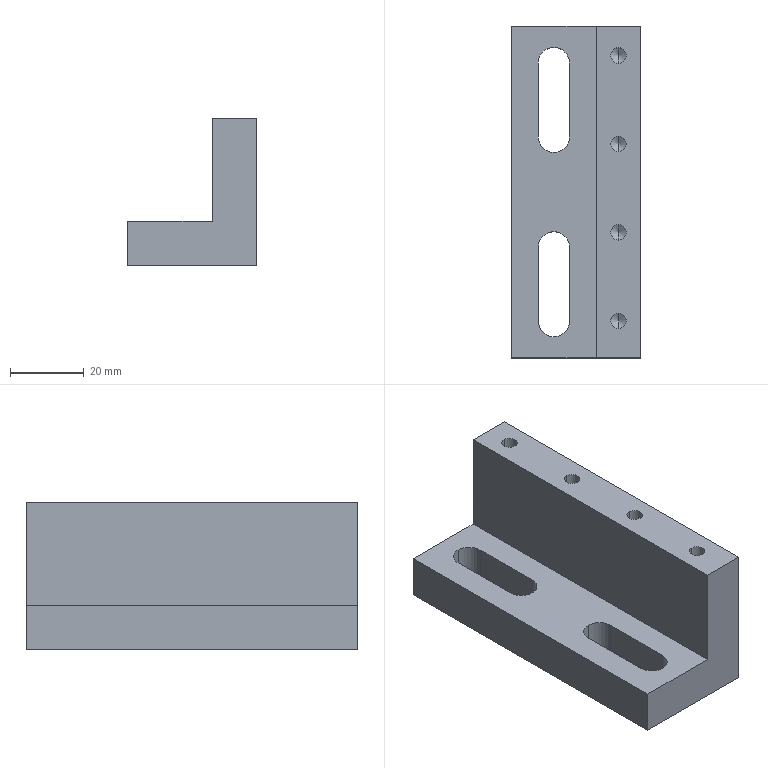Component | SolidWorks | DC-024-05-1 | 1 solid | 34 faces | box 35 x 90 x 40 mm | volume 61888 mm3 | cylinder 14 | plane 12 | cone 8 | commonest cylinder face diameters 4.2 x8 8.5 x6
build123d program:
from build123d import *

# Parameters (mm, degrees)
BOSS_EXTRUDE1_DEPTH   = 45
CUT_EXTRUDE1_DEPTH    = 80
M5_TAPPED_HOLE1_D     = 4.2
M5_TAPPED_HOLE1_DEPTH = 12.4
M5_TAPPED_HOLE1_TIP   = 1.262


with BuildPart() as part:
    # Sketch1 → Boss-Extrude1 (new, symmetric)
    with BuildSketch(Plane.XY):
        Polygon((0, 35), (0, 0), (40, 0), (40, 12), (12, 12), (12, 35), align=None)
    extrude(amount=BOSS_EXTRUDE1_DEPTH, both=True)

    # Sketch2 → Cut-Extrude1 (cut)
    with BuildSketch(Plane(origin=(12, 0, 0), x_dir=(0, 0, -1), z_dir=(1, 0, 0))):
        with BuildLine():
            Line((35, 19.25), (15, 19.25))
            ThreePointArc((15, 19.25), (10.75, 23.5), (15, 27.75))
            Line((15, 27.75), (35, 27.75))
            ThreePointArc((35, 27.75), (39.25, 23.5), (35, 19.25))
        make_face()
        with BuildLine():
            Line((-35, 19.25), (-15, 19.25))
            ThreePointArc((-15, 19.25), (-10.75, 23.5), (-15, 27.75))
            Line((-15, 27.75), (-35, 27.75))
            ThreePointArc((-35, 27.75), (-39.25, 23.5), (-35, 19.25))
        make_face()
    extrude(amount=-CUT_EXTRUDE1_DEPTH, mode=Mode.SUBTRACT)

    # M5 Tapped Hole1
    with Locations(Plane(origin=(40, 0, 0), x_dir=(0, 0, -1), z_dir=(1, 0, 0))):
        with Locations((37, 6), (13, 6), (-11, 6), (-35, 6)):
            Hole(M5_TAPPED_HOLE1_D / 2, depth=M5_TAPPED_HOLE1_DEPTH)
            with Locations((0, 0, -(M5_TAPPED_HOLE1_DEPTH + M5_TAPPED_HOLE1_TIP / 2))):  # 118° drill point
                Cone(0, M5_TAPPED_HOLE1_D / 2, M5_TAPPED_HOLE1_TIP, mode=Mode.SUBTRACT)


solid = part.part

# Placed as in the assembly
solid = solid.moved(Location((-78.633, -394.091, 13), (90, 0, 90)))
STEP:
#1=CARTESIAN_POINT('',(-3.332,-14.141,1.598));
#2=VERTEX_POINT('',#1);
#3=CARTESIAN_POINT('',(-3.332,-13.976,1.598));
#4=VERTEX_POINT('',#3);
#5=CARTESIAN_POINT('',(-3.332,-14.059,1.598));
#6=DIRECTION('',(-0.,-0.,1.));
#7=DIRECTION('',(0.,1.,0.));
#8=AXIS2_PLACEMENT_3D('',#5,#6,#7);
#9=CIRCLE('',#8,0.08268);
#10=EDGE_CURVE('',#2,#4,#9,.T.);
#11=ORIENTED_EDGE('',*,*,#10,.F.);
#12=CARTESIAN_POINT('',(-3.332,-14.141,2.087));
#13=VERTEX_POINT('',#12);
#14=CARTESIAN_POINT('',(-3.332,-14.141,2.087));
#15=DIRECTION('',(-0.,-0.,1.));
#16=VECTOR('',#15,39.37);
#17=LINE('',#14,#16);
#18=EDGE_CURVE('',#2,#13,#17,.T.);
#19=ORIENTED_EDGE('',*,*,#18,.T.);
#20=CARTESIAN_POINT('',(-3.332,-13.976,2.087));
#21=VERTEX_POINT('',#20);
#22=CARTESIAN_POINT('',(-3.332,-14.059,2.087));
#23=DIRECTION('',(-0.,-0.,1.));
#24=DIRECTION('',(0.,1.,0.));
#25=AXIS2_PLACEMENT_3D('',#22,#23,#24);
#26=CIRCLE('',#25,0.08268);
#27=EDGE_CURVE('',#13,#21,#26,.T.);
#28=ORIENTED_EDGE('',*,*,#27,.T.);
#29=CARTESIAN_POINT('',(-3.332,-13.976,2.087));
#30=DIRECTION('',(-0.,-0.,1.));
#31=VECTOR('',#30,39.37);
#32=LINE('',#29,#31);
#33=EDGE_CURVE('',#4,#21,#32,.T.);
#34=ORIENTED_EDGE('',*,*,#33,.F.);
#35=EDGE_LOOP('',(#11,#19,#28,#34));
#36=FACE_OUTER_BOUND('',#35,.T.);
#37=CARTESIAN_POINT('',(-3.332,-14.059,2.087));
#38=DIRECTION('',(-0.,-0.,1.));
#39=DIRECTION('',(0.,1.,0.));
#40=AXIS2_PLACEMENT_3D('',#37,#38,#39);
#41=CYLINDRICAL_SURFACE('',#40,0.08268);
#42=ADVANCED_FACE('',(#36),#41,.F.);
#43=CARTESIAN_POINT('',(-3.332,-14.059,1.549));
#44=VERTEX_POINT('',#43);
#45=CARTESIAN_POINT('',(-3.332,-13.976,1.598));
#46=DIRECTION('',(-0.,0.8572,0.515));
#47=VECTOR('',#46,39.37);
#48=LINE('',#45,#47);
#49=EDGE_CURVE('',#44,#4,#48,.T.);
#50=ORIENTED_EDGE('',*,*,#49,.F.);
#51=CARTESIAN_POINT('',(-3.332,-14.141,1.598));
#52=DIRECTION('',(0.,-0.8572,0.515));
#53=VECTOR('',#52,39.37);
#54=LINE('',#51,#53);
#55=EDGE_CURVE('',#44,#2,#54,.T.);
#56=ORIENTED_EDGE('',*,*,#55,.T.);
#57=ORIENTED_EDGE('',*,*,#10,.T.);
#58=EDGE_LOOP('',(#50,#56,#57));
#59=FACE_OUTER_BOUND('',#58,.T.);
#60=CARTESIAN_POINT('',(-3.332,-14.059,1.598));
#61=DIRECTION('',(-0.,-0.,1.));
#62=DIRECTION('',(0.,1.,0.));
#63=AXIS2_PLACEMENT_3D('',#60,#61,#62);
#64=CONICAL_SURFACE('',#63,0.08268,1.03);
#65=ADVANCED_FACE('',(#59),#64,.F.);
#66=CARTESIAN_POINT('',(-3.332,-15.086,1.598));
#67=VERTEX_POINT('',#66);
#68=CARTESIAN_POINT('',(-3.332,-14.921,1.598));
#69=VERTEX_POINT('',#68);
#70=CARTESIAN_POINT('',(-3.332,-15.004,1.598));
#71=DIRECTION('',(-0.,-0.,1.));
#72=DIRECTION('',(0.,1.,0.));
#73=AXIS2_PLACEMENT_3D('',#70,#71,#72);
#74=CIRCLE('',#73,0.08268);
#75=EDGE_CURVE('',#67,#69,#74,.T.);
#76=ORIENTED_EDGE('',*,*,#75,.F.);
#77=CARTESIAN_POINT('',(-3.332,-15.086,2.087));
#78=VERTEX_POINT('',#77);
#79=CARTESIAN_POINT('',(-3.332,-15.086,2.087));
#80=DIRECTION('',(-0.,-0.,1.));
#81=VECTOR('',#80,39.37);
#82=LINE('',#79,#81);
#83=EDGE_CURVE('',#67,#78,#82,.T.);
#84=ORIENTED_EDGE('',*,*,#83,.T.);
#85=CARTESIAN_POINT('',(-3.332,-14.921,2.087));
#86=VERTEX_POINT('',#85);
#87=CARTESIAN_POINT('',(-3.332,-15.004,2.087));
#88=DIRECTION('',(-0.,-0.,1.));
#89=DIRECTION('',(0.,1.,0.));
#90=AXIS2_PLACEMENT_3D('',#87,#88,#89);
#91=CIRCLE('',#90,0.08268);
#92=EDGE_CURVE('',#78,#86,#91,.T.);
#93=ORIENTED_EDGE('',*,*,#92,.T.);
#94=CARTESIAN_POINT('',(-3.332,-14.921,2.087));
#95=DIRECTION('',(-0.,-0.,1.));
#96=VECTOR('',#95,39.37);
#97=LINE('',#94,#96);
#98=EDGE_CURVE('',#69,#86,#97,.T.);
#99=ORIENTED_EDGE('',*,*,#98,.F.);
#100=EDGE_LOOP('',(#76,#84,#93,#99));
#101=FACE_OUTER_BOUND('',#100,.T.);
#102=CARTESIAN_POINT('',(-3.332,-15.004,2.087));
#103=DIRECTION('',(-0.,-0.,1.));
#104=DIRECTION('',(0.,1.,0.));
#105=AXIS2_PLACEMENT_3D('',#102,#103,#104);
#106=CYLINDRICAL_SURFACE('',#105,0.08268);
#107=ADVANCED_FACE('',(#101),#106,.F.);
#108=CARTESIAN_POINT('',(-3.332,-15.004,1.549));
#109=VERTEX_POINT('',#108);
#110=CARTESIAN_POINT('',(-3.332,-14.921,1.598));
#111=DIRECTION('',(-0.,0.8572,0.515));
#112=VECTOR('',#111,39.37);
#113=LINE('',#110,#112);
#114=EDGE_CURVE('',#109,#69,#113,.T.);
#115=ORIENTED_EDGE('',*,*,#114,.F.);
#116=CARTESIAN_POINT('',(-3.332,-15.086,1.598));
#117=DIRECTION('',(0.,-0.8572,0.515));
#118=VECTOR('',#117,39.37);
#119=LINE('',#116,#118);
#120=EDGE_CURVE('',#109,#67,#119,.T.);
#121=ORIENTED_EDGE('',*,*,#120,.T.);
#122=ORIENTED_EDGE('',*,*,#75,.T.);
#123=EDGE_LOOP('',(#115,#121,#122));
#124=FACE_OUTER_BOUND('',#123,.T.);
#125=CARTESIAN_POINT('',(-3.332,-15.004,1.598));
#126=DIRECTION('',(-0.,-0.,1.));
#127=DIRECTION('',(0.,1.,0.));
#128=AXIS2_PLACEMENT_3D('',#125,#126,#127);
#129=CONICAL_SURFACE('',#128,0.08268,1.03);
#130=ADVANCED_FACE('',(#124),#129,.F.);
#131=CARTESIAN_POINT('',(-3.332,-16.031,1.598));
#132=VERTEX_POINT('',#131);
#133=CARTESIAN_POINT('',(-3.332,-15.866,1.598));
#134=VERTEX_POINT('',#133);
#135=CARTESIAN_POINT('',(-3.332,-15.948,1.598));
#136=DIRECTION('',(-0.,-0.,1.));
#137=DIRECTION('',(0.,1.,0.));
#138=AXIS2_PLACEMENT_3D('',#135,#136,#137);
#139=CIRCLE('',#138,0.08268);
#140=EDGE_CURVE('',#132,#134,#139,.T.);
#141=ORIENTED_EDGE('',*,*,#140,.F.);
#142=CARTESIAN_POINT('',(-3.332,-16.031,2.087));
#143=VERTEX_POINT('',#142);
#144=CARTESIAN_POINT('',(-3.332,-16.031,2.087));
#145=DIRECTION('',(-0.,-0.,1.));
#146=VECTOR('',#145,39.37);
#147=LINE('',#144,#146);
#148=EDGE_CURVE('',#132,#143,#147,.T.);
#149=ORIENTED_EDGE('',*,*,#148,.T.);
#150=CARTESIAN_POINT('',(-3.332,-15.866,2.087));
#151=VERTEX_POINT('',#150);
#152=CARTESIAN_POINT('',(-3.332,-15.948,2.087));
#153=DIRECTION('',(-0.,-0.,1.));
#154=DIRECTION('',(0.,1.,0.));
#155=AXIS2_PLACEMENT_3D('',#152,#153,#154);
#156=CIRCLE('',#155,0.08268);
#157=EDGE_CURVE('',#143,#151,#156,.T.);
#158=ORIENTED_EDGE('',*,*,#157,.T.);
#159=CARTESIAN_POINT('',(-3.332,-15.866,2.087));
#160=DIRECTION('',(-0.,-0.,1.));
#161=VECTOR('',#160,39.37);
#162=LINE('',#159,#161);
#163=EDGE_CURVE('',#134,#151,#162,.T.);
#164=ORIENTED_EDGE('',*,*,#163,.F.);
#165=EDGE_LOOP('',(#141,#149,#158,#164));
#166=FACE_OUTER_BOUND('',#165,.T.);
#167=CARTESIAN_POINT('',(-3.332,-15.948,2.087));
#168=DIRECTION('',(-0.,-0.,1.));
#169=DIRECTION('',(0.,1.,0.));
#170=AXIS2_PLACEMENT_3D('',#167,#168,#169);
#171=CYLINDRICAL_SURFACE('',#170,0.08268);
#172=ADVANCED_FACE('',(#166),#171,.F.);
#173=CARTESIAN_POINT('',(-3.332,-15.948,1.549));
#174=VERTEX_POINT('',#173);
#175=CARTESIAN_POINT('',(-3.332,-15.866,1.598));
#176=DIRECTION('',(-0.,0.8572,0.515));
#177=VECTOR('',#176,39.37);
#178=LINE('',#175,#177);
#179=EDGE_CURVE('',#174,#134,#178,.T.);
#180=ORIENTED_EDGE('',*,*,#179,.F.);
#181=CARTESIAN_POINT('',(-3.332,-16.031,1.598));
#182=DIRECTION('',(0.,-0.8572,0.515));
#183=VECTOR('',#182,39.37);
#184=LINE('',#181,#183);
#185=EDGE_CURVE('',#174,#132,#184,.T.);
#186=ORIENTED_EDGE('',*,*,#185,.T.);
#187=ORIENTED_EDGE('',*,*,#140,.T.);
#188=EDGE_LOOP('',(#180,#186,#187));
#189=FACE_OUTER_BOUND('',#188,.T.);
#190=CARTESIAN_POINT('',(-3.332,-15.948,1.598));
#191=DIRECTION('',(-0.,-0.,1.));
#192=DIRECTION('',(0.,1.,0.));
#193=AXIS2_PLACEMENT_3D('',#190,#191,#192);
#194=CONICAL_SURFACE('',#193,0.08268,1.03);
#195=ADVANCED_FACE('',(#189),#194,.F.);
#196=CARTESIAN_POINT('',(-3.332,-16.976,1.598));
#197=VERTEX_POINT('',#196);
#198=CARTESIAN_POINT('',(-3.332,-16.811,1.598));
#199=VERTEX_POINT('',#198);
#200=CARTESIAN_POINT('',(-3.332,-16.893,1.598));
#201=DIRECTION('',(-0.,-0.,1.));
#202=DIRECTION('',(0.,1.,0.));
#203=AXIS2_PLACEMENT_3D('',#200,#201,#202);
#204=CIRCLE('',#203,0.08268);
#205=EDGE_CURVE('',#197,#199,#204,.T.);
#206=ORIENTED_EDGE('',*,*,#205,.F.);
#207=CARTESIAN_POINT('',(-3.332,-16.976,2.087));
#208=VERTEX_POINT('',#207);
#209=CARTESIAN_POINT('',(-3.332,-16.976,2.087));
#210=DIRECTION('',(-0.,-0.,1.));
#211=VECTOR('',#210,39.37);
#212=LINE('',#209,#211);
#213=EDGE_CURVE('',#197,#208,#212,.T.);
#214=ORIENTED_EDGE('',*,*,#213,.T.);
#215=CARTESIAN_POINT('',(-3.332,-16.811,2.087));
#216=VERTEX_POINT('',#215);
#217=CARTESIAN_POINT('',(-3.332,-16.893,2.087));
#218=DIRECTION('',(-0.,-0.,1.));
#219=DIRECTION('',(0.,1.,0.));
#220=AXIS2_PLACEMENT_3D('',#217,#218,#219);
#221=CIRCLE('',#220,0.08268);
#222=EDGE_CURVE('',#208,#216,#221,.T.);
#223=ORIENTED_EDGE('',*,*,#222,.T.);
#224=CARTESIAN_POINT('',(-3.332,-16.811,2.087));
#225=DIRECTION('',(-0.,-0.,1.));
#226=VECTOR('',#225,39.37);
#227=LINE('',#224,#226);
#228=EDGE_CURVE('',#199,#216,#227,.T.);
#229=ORIENTED_EDGE('',*,*,#228,.F.);
#230=EDGE_LOOP('',(#206,#214,#223,#229));
#231=FACE_OUTER_BOUND('',#230,.T.);
#232=CARTESIAN_POINT('',(-3.332,-16.893,2.087));
#233=DIRECTION('',(-0.,-0.,1.));
#234=DIRECTION('',(0.,1.,0.));
#235=AXIS2_PLACEMENT_3D('',#232,#233,#234);
#236=CYLINDRICAL_SURFACE('',#235,0.08268);
#237=ADVANCED_FACE('',(#231),#236,.F.);
#238=CARTESIAN_POINT('',(-3.332,-16.893,1.549));
#239=VERTEX_POINT('',#238);
#240=CARTESIAN_POINT('',(-3.332,-16.811,1.598));
#241=DIRECTION('',(-0.,0.8572,0.515));
#242=VECTOR('',#241,39.37);
#243=LINE('',#240,#242);
#244=EDGE_CURVE('',#239,#199,#243,.T.);
#245=ORIENTED_EDGE('',*,*,#244,.F.);
#246=CARTESIAN_POINT('',(-3.332,-16.976,1.598));
#247=DIRECTION('',(0.,-0.8572,0.515));
#248=VECTOR('',#247,39.37);
#249=LINE('',#246,#248);
#250=EDGE_CURVE('',#239,#197,#249,.T.);
#251=ORIENTED_EDGE('',*,*,#250,.T.);
#252=ORIENTED_EDGE('',*,*,#205,.T.);
#253=EDGE_LOOP('',(#245,#251,#252));
#254=FACE_OUTER_BOUND('',#253,.T.);
#255=CARTESIAN_POINT('',(-3.332,-16.893,1.598));
#256=DIRECTION('',(-0.,-0.,1.));
#257=DIRECTION('',(0.,1.,0.));
#258=AXIS2_PLACEMENT_3D('',#255,#256,#257);
#259=CONICAL_SURFACE('',#258,0.08268,1.03);
#260=ADVANCED_FACE('',(#254),#259,.F.);
#261=CARTESIAN_POINT('',(-4.021,-13.97,0.5118));
#262=VERTEX_POINT('',#261);
#263=CARTESIAN_POINT('',(-4.188,-14.137,0.5118));
#264=VERTEX_POINT('',#263);
#265=CARTESIAN_POINT('',(-4.021,-14.137,0.5118));
#266=DIRECTION('',(-0.,-0.,1.));
#267=DIRECTION('',(-1.,0.,0.));
#268=AXIS2_PLACEMENT_3D('',#265,#266,#267);
#269=CIRCLE('',#268,0.1673);
#270=EDGE_CURVE('',#262,#264,#269,.T.);
#271=ORIENTED_EDGE('',*,*,#270,.F.);
#272=CARTESIAN_POINT('',(-4.021,-13.97,0.9843));
#273=VERTEX_POINT('',#272);
#274=CARTESIAN_POINT('',(-4.021,-13.97,-2.165));
#275=DIRECTION('',(-0.,-0.,1.));
#276=VECTOR('',#275,39.37);
#277=LINE('',#274,#276);
#278=EDGE_CURVE('',#262,#273,#277,.T.);
#279=ORIENTED_EDGE('',*,*,#278,.T.);
#280=CARTESIAN_POINT('',(-4.188,-14.137,0.9843));
#281=VERTEX_POINT('',#280);
#282=CARTESIAN_POINT('',(-4.021,-14.137,0.9843));
#283=DIRECTION('',(-0.,-0.,1.));
#284=DIRECTION('',(0.,1.,0.));
#285=AXIS2_PLACEMENT_3D('',#282,#283,#284);
#286=CIRCLE('',#285,0.1673);
#287=EDGE_CURVE('',#273,#281,#286,.T.);
#288=ORIENTED_EDGE('',*,*,#287,.T.);
#289=CARTESIAN_POINT('',(-4.188,-14.137,-2.165));
#290=DIRECTION('',(-0.,-0.,1.));
#291=VECTOR('',#290,39.37);
#292=LINE('',#289,#291);
#293=EDGE_CURVE('',#264,#281,#292,.T.);
#294=ORIENTED_EDGE('',*,*,#293,.F.);
#295=EDGE_LOOP('',(#271,#279,#288,#294));
#296=FACE_OUTER_BOUND('',#295,.T.);
#297=CARTESIAN_POINT('',(-4.021,-14.137,-2.165));
#298=DIRECTION('',(-0.,-0.,1.));
#299=DIRECTION('',(0.,1.,0.));
#300=AXIS2_PLACEMENT_3D('',#297,#298,#299);
#301=CYLINDRICAL_SURFACE('',#300,0.1673);
#302=ADVANCED_FACE('',(#296),#301,.F.);
#303=CARTESIAN_POINT('',(-4.021,-15.939,0.5118));
#304=VERTEX_POINT('',#303);
#305=CARTESIAN_POINT('',(-4.188,-16.106,0.5118));
#306=VERTEX_POINT('',#305);
#307=CARTESIAN_POINT('',(-4.021,-16.106,0.5118));
#308=DIRECTION('',(-0.,-0.,1.));
#309=DIRECTION('',(-1.,0.,0.));
#310=AXIS2_PLACEMENT_3D('',#307,#308,#309);
#311=CIRCLE('',#310,0.1673);
#312=EDGE_CURVE('',#304,#306,#311,.T.);
#313=ORIENTED_EDGE('',*,*,#312,.F.);
#314=CARTESIAN_POINT('',(-4.021,-15.939,0.9843));
#315=VERTEX_POINT('',#314);
#316=CARTESIAN_POINT('',(-4.021,-15.939,-2.165));
#317=DIRECTION('',(-0.,-0.,1.));
#318=VECTOR('',#317,39.37);
#319=LINE('',#316,#318);
#320=EDGE_CURVE('',#304,#315,#319,.T.);
#321=ORIENTED_EDGE('',*,*,#320,.T.);
#322=CARTESIAN_POINT('',(-4.188,-16.106,0.9843));
#323=VERTEX_POINT('',#322);
#324=CARTESIAN_POINT('',(-4.021,-16.106,0.9843));
#325=DIRECTION('',(-0.,-0.,1.));
#326=DIRECTION('',(0.,-1.,0.));
#327=AXIS2_PLACEMENT_3D('',#324,#325,#326);
#328=CIRCLE('',#327,0.1673);
#329=EDGE_CURVE('',#315,#323,#328,.T.);
#330=ORIENTED_EDGE('',*,*,#329,.T.);
#331=CARTESIAN_POINT('',(-4.188,-16.106,-2.165));
#332=DIRECTION('',(-0.,-0.,1.));
#333=VECTOR('',#332,39.37);
#334=LINE('',#331,#333);
#335=EDGE_CURVE('',#306,#323,#334,.T.);
#336=ORIENTED_EDGE('',*,*,#335,.F.);
#337=EDGE_LOOP('',(#313,#321,#330,#336));
#338=FACE_OUTER_BOUND('',#337,.T.);
#339=CARTESIAN_POINT('',(-4.021,-16.106,-2.165));
#340=DIRECTION('',(-0.,-0.,1.));
#341=DIRECTION('',(0.,1.,0.));
#342=AXIS2_PLACEMENT_3D('',#339,#340,#341);
#343=CYLINDRICAL_SURFACE('',#342,0.1673);
#344=ADVANCED_FACE('',(#338),#343,.F.);
#345=CARTESIAN_POINT('',(-4.474,-13.744,0.9843));
#346=VERTEX_POINT('',#345);
#347=CARTESIAN_POINT('',(-4.474,-13.744,0.5118));
#348=VERTEX_POINT('',#347);
#349=CARTESIAN_POINT('',(-4.474,-13.744,0.5118));
#350=DIRECTION('',(0.,0.,-1.));
#351=VECTOR('',#350,39.37);
#352=LINE('',#349,#351);
#353=EDGE_CURVE('',#346,#348,#352,.T.);
#354=ORIENTED_EDGE('',*,*,#353,.T.);
#355=CARTESIAN_POINT('',(-4.474,-17.287,0.5118));
#356=VERTEX_POINT('',#355);
#357=CARTESIAN_POINT('',(-4.474,-17.287,0.5118));
#358=DIRECTION('',(-0.,1.,0.));
#359=VECTOR('',#358,39.37);
#360=LINE('',#357,#359);
#361=EDGE_CURVE('',#356,#348,#360,.T.);
#362=ORIENTED_EDGE('',*,*,#361,.F.);
#363=CARTESIAN_POINT('',(-4.474,-17.287,0.9843));
#364=VERTEX_POINT('',#363);
#365=CARTESIAN_POINT('',(-4.474,-17.287,0.5118));
#366=DIRECTION('',(0.,0.,-1.));
#367=VECTOR('',#366,39.37);
#368=LINE('',#365,#367);
#369=EDGE_CURVE('',#364,#356,#368,.T.);
#370=ORIENTED_EDGE('',*,*,#369,.F.);
#371=CARTESIAN_POINT('',(-4.474,-17.287,0.9843));
#372=DIRECTION('',(-0.,1.,0.));
#373=VECTOR('',#372,39.37);
#374=LINE('',#371,#373);
#375=EDGE_CURVE('',#364,#346,#374,.T.);
#376=ORIENTED_EDGE('',*,*,#375,.T.);
#377=EDGE_LOOP('',(#354,#362,#370,#376));
#378=FACE_OUTER_BOUND('',#377,.T.);
#379=CARTESIAN_POINT('',(-4.474,-17.287,0.5118));
#380=DIRECTION('',(1.,0.,0.));
#381=DIRECTION('',(-0.,1.,0.));
#382=AXIS2_PLACEMENT_3D('',#379,#380,#381);
#383=PLANE('',#382);
#384=ADVANCED_FACE('',(#378),#383,.F.);
#385=CARTESIAN_POINT('',(-3.854,-14.925,0.5118));
#386=VERTEX_POINT('',#385);
#387=CARTESIAN_POINT('',(-3.854,-14.137,0.5118));
#388=VERTEX_POINT('',#387);
#389=CARTESIAN_POINT('',(-3.854,-17.287,0.5118));
#390=DIRECTION('',(-0.,1.,0.));
#391=VECTOR('',#390,39.37);
#392=LINE('',#389,#391);
#393=EDGE_CURVE('',#386,#388,#392,.T.);
#394=ORIENTED_EDGE('',*,*,#393,.T.);
#395=CARTESIAN_POINT('',(-4.021,-14.137,0.5118));
#396=DIRECTION('',(-0.,-0.,1.));
#397=DIRECTION('',(-1.,0.,0.));
#398=AXIS2_PLACEMENT_3D('',#395,#396,#397);
#399=CIRCLE('',#398,0.1673);
#400=EDGE_CURVE('',#388,#262,#399,.T.);
#401=ORIENTED_EDGE('',*,*,#400,.T.);
#402=ORIENTED_EDGE('',*,*,#270,.T.);
#403=CARTESIAN_POINT('',(-4.188,-14.925,0.5118));
#404=VERTEX_POINT('',#403);
#405=CARTESIAN_POINT('',(-4.188,-17.287,0.5118));
#406=DIRECTION('',(0.,-1.,0.));
#407=VECTOR('',#406,39.37);
#408=LINE('',#405,#407);
#409=EDGE_CURVE('',#264,#404,#408,.T.);
#410=ORIENTED_EDGE('',*,*,#409,.T.);
#411=CARTESIAN_POINT('',(-4.021,-14.925,0.5118));
#412=DIRECTION('',(-0.,-0.,1.));
#413=DIRECTION('',(-1.,0.,0.));
#414=AXIS2_PLACEMENT_3D('',#411,#412,#413);
#415=CIRCLE('',#414,0.1673);
#416=EDGE_CURVE('',#404,#386,#415,.T.);
#417=ORIENTED_EDGE('',*,*,#416,.T.);
#418=EDGE_LOOP('',(#394,#401,#402,#410,#417));
#419=FACE_BOUND('',#418,.T.);
#420=CARTESIAN_POINT('',(-4.188,-16.893,0.5118));
#421=VERTEX_POINT('',#420);
#422=CARTESIAN_POINT('',(-4.188,-17.287,0.5118));
#423=DIRECTION('',(0.,-1.,0.));
#424=VECTOR('',#423,39.37);
#425=LINE('',#422,#424);
#426=EDGE_CURVE('',#306,#421,#425,.T.);
#427=ORIENTED_EDGE('',*,*,#426,.T.);
#428=CARTESIAN_POINT('',(-3.854,-16.893,0.5118));
#429=VERTEX_POINT('',#428);
#430=CARTESIAN_POINT('',(-4.021,-16.893,0.5118));
#431=DIRECTION('',(-0.,-0.,1.));
#432=DIRECTION('',(-1.,0.,0.));
#433=AXIS2_PLACEMENT_3D('',#430,#431,#432);
#434=CIRCLE('',#433,0.1673);
#435=EDGE_CURVE('',#421,#429,#434,.T.);
#436=ORIENTED_EDGE('',*,*,#435,.T.);
#437=CARTESIAN_POINT('',(-3.854,-16.106,0.5118));
#438=VERTEX_POINT('',#437);
#439=CARTESIAN_POINT('',(-3.854,-17.287,0.5118));
#440=DIRECTION('',(-0.,1.,0.));
#441=VECTOR('',#440,39.37);
#442=LINE('',#439,#441);
#443=EDGE_CURVE('',#429,#438,#442,.T.);
#444=ORIENTED_EDGE('',*,*,#443,.T.);
#445=CARTESIAN_POINT('',(-4.021,-16.106,0.5118));
#446=DIRECTION('',(-0.,-0.,1.));
#447=DIRECTION('',(-1.,0.,0.));
#448=AXIS2_PLACEMENT_3D('',#445,#446,#447);
#449=CIRCLE('',#448,0.1673);
#450=EDGE_CURVE('',#438,#304,#449,.T.);
#451=ORIENTED_EDGE('',*,*,#450,.T.);
#452=ORIENTED_EDGE('',*,*,#312,.T.);
#453=EDGE_LOOP('',(#427,#436,#444,#451,#452));
#454=FACE_BOUND('',#453,.T.);
#455=CARTESIAN_POINT('',(-3.096,-13.744,0.5118));
#456=VERTEX_POINT('',#455);
#457=CARTESIAN_POINT('',(-4.474,-13.744,0.5118));
#458=DIRECTION('',(1.,0.,0.));
#459=VECTOR('',#458,39.37);
#460=LINE('',#457,#459);
#461=EDGE_CURVE('',#348,#456,#460,.T.);
#462=ORIENTED_EDGE('',*,*,#461,.T.);
#463=CARTESIAN_POINT('',(-3.096,-17.287,0.5118));
#464=VERTEX_POINT('',#463);
#465=CARTESIAN_POINT('',(-3.096,-17.287,0.5118));
#466=DIRECTION('',(-0.,1.,0.));
#467=VECTOR('',#466,39.37);
#468=LINE('',#465,#467);
#469=EDGE_CURVE('',#464,#456,#468,.T.);
#470=ORIENTED_EDGE('',*,*,#469,.F.);
#471=CARTESIAN_POINT('',(-4.474,-17.287,0.5118));
#472=DIRECTION('',(1.,0.,0.));
#473=VECTOR('',#472,39.37);
#474=LINE('',#471,#473);
#475=EDGE_CURVE('',#356,#464,#474,.T.);
#476=ORIENTED_EDGE('',*,*,#475,.F.);
#477=ORIENTED_EDGE('',*,*,#361,.T.);
#478=EDGE_LOOP('',(#462,#470,#476,#477));
#479=FACE_OUTER_BOUND('',#478,.T.);
#480=CARTESIAN_POINT('',(-4.474,-17.287,0.5118));
#481=DIRECTION('',(-0.,-0.,1.));
#482=DIRECTION('',(-1.,-0.,-0.));
#483=AXIS2_PLACEMENT_3D('',#480,#481,#482);
#484=PLANE('',#483);
#485=ADVANCED_FACE('',(#419,#454,#479),#484,.F.);
#486=CARTESIAN_POINT('',(-3.096,-13.744,2.087));
#487=VERTEX_POINT('',#486);
#488=CARTESIAN_POINT('',(-3.096,-13.744,0.5118));
#489=DIRECTION('',(-0.,-0.,1.));
#490=VECTOR('',#489,39.37);
#491=LINE('',#488,#490);
#492=EDGE_CURVE('',#456,#487,#491,.T.);
#493=ORIENTED_EDGE('',*,*,#492,.T.);
#494=CARTESIAN_POINT('',(-3.096,-17.287,2.087));
#495=VERTEX_POINT('',#494);
#496=CARTESIAN_POINT('',(-3.096,-17.287,2.087));
#497=DIRECTION('',(-0.,1.,0.));
#498=VECTOR('',#497,39.37);
#499=LINE('',#496,#498);
#500=EDGE_CURVE('',#495,#487,#499,.T.);
#501=ORIENTED_EDGE('',*,*,#500,.F.);
#502=CARTESIAN_POINT('',(-3.096,-17.287,0.5118));
#503=DIRECTION('',(-0.,-0.,1.));
#504=VECTOR('',#503,39.37);
#505=LINE('',#502,#504);
#506=EDGE_CURVE('',#464,#495,#505,.T.);
#507=ORIENTED_EDGE('',*,*,#506,.F.);
#508=ORIENTED_EDGE('',*,*,#469,.T.);
#509=EDGE_LOOP('',(#493,#501,#507,#508));
#510=FACE_OUTER_BOUND('',#509,.T.);
#511=CARTESIAN_POINT('',(-3.096,-17.287,0.5118));
#512=DIRECTION('',(-1.,-0.,-0.));
#513=DIRECTION('',(0.,-1.,0.));
#514=AXIS2_PLACEMENT_3D('',#511,#512,#513);
#515=PLANE('',#514);
#516=ADVANCED_FACE('',(#510),#515,.F.);
#517=CARTESIAN_POINT('',(-3.332,-14.059,2.087));
#518=DIRECTION('',(-0.,-0.,1.));
#519=DIRECTION('',(0.,1.,0.));
#520=AXIS2_PLACEMENT_3D('',#517,#518,#519);
#521=CIRCLE('',#520,0.08268);
#522=EDGE_CURVE('',#21,#13,#521,.T.);
#523=ORIENTED_EDGE('',*,*,#522,.F.);
#524=ORIENTED_EDGE('',*,*,#27,.F.);
#525=EDGE_LOOP('',(#523,#524));
#526=FACE_BOUND('',#525,.T.);
#527=CARTESIAN_POINT('',(-3.332,-15.004,2.087));
#528=DIRECTION('',(-0.,-0.,1.));
#529=DIRECTION('',(0.,1.,0.));
#530=AXIS2_PLACEMENT_3D('',#527,#528,#529);
#531=CIRCLE('',#530,0.08268);
#532=EDGE_CURVE('',#86,#78,#531,.T.);
#533=ORIENTED_EDGE('',*,*,#532,.F.);
#534=ORIENTED_EDGE('',*,*,#92,.F.);
#535=EDGE_LOOP('',(#533,#534));
#536=FACE_BOUND('',#535,.T.);
#537=CARTESIAN_POINT('',(-3.332,-15.948,2.087));
#538=DIRECTION('',(-0.,-0.,1.));
#539=DIRECTION('',(0.,1.,0.));
#540=AXIS2_PLACEMENT_3D('',#537,#538,#539);
#541=CIRCLE('',#540,0.08268);
#542=EDGE_CURVE('',#151,#143,#541,.T.);
#543=ORIENTED_EDGE('',*,*,#542,.F.);
#544=ORIENTED_EDGE('',*,*,#157,.F.);
#545=EDGE_LOOP('',(#543,#544));
#546=FACE_BOUND('',#545,.T.);
#547=CARTESIAN_POINT('',(-3.332,-16.893,2.087));
#548=DIRECTION('',(-0.,-0.,1.));
#549=DIRECTION('',(0.,1.,0.));
#550=AXIS2_PLACEMENT_3D('',#547,#548,#549);
#551=CIRCLE('',#550,0.08268);
#552=EDGE_CURVE('',#216,#208,#551,.T.);
#553=ORIENTED_EDGE('',*,*,#552,.F.);
#554=ORIENTED_EDGE('',*,*,#222,.F.);
#555=EDGE_LOOP('',(#553,#554));
#556=FACE_BOUND('',#555,.T.);
#557=CARTESIAN_POINT('',(-3.568,-13.744,2.087));
#558=VERTEX_POINT('',#557);
#559=CARTESIAN_POINT('',(-3.568,-13.744,2.087));
#560=DIRECTION('',(-1.,-0.,-0.));
#561=VECTOR('',#560,39.37);
#562=LINE('',#559,#561);
#563=EDGE_CURVE('',#487,#558,#562,.T.);
#564=ORIENTED_EDGE('',*,*,#563,.T.);
#565=CARTESIAN_POINT('',(-3.568,-17.287,2.087));
#566=VERTEX_POINT('',#565);
#567=CARTESIAN_POINT('',(-3.568,-17.287,2.087));
#568=DIRECTION('',(-0.,1.,0.));
#569=VECTOR('',#568,39.37);
#570=LINE('',#567,#569);
#571=EDGE_CURVE('',#566,#558,#570,.T.);
#572=ORIENTED_EDGE('',*,*,#571,.F.);
#573=CARTESIAN_POINT('',(-3.568,-17.287,2.087));
#574=DIRECTION('',(-1.,-0.,-0.));
#575=VECTOR('',#574,39.37);
#576=LINE('',#573,#575);
#577=EDGE_CURVE('',#495,#566,#576,.T.);
#578=ORIENTED_EDGE('',*,*,#577,.F.);
#579=ORIENTED_EDGE('',*,*,#500,.T.);
#580=EDGE_LOOP('',(#564,#572,#578,#579));
#581=FACE_OUTER_BOUND('',#580,.T.);
#582=CARTESIAN_POINT('',(-3.568,-17.287,2.087));
#583=DIRECTION('',(0.,0.,-1.));
#584=DIRECTION('',(0.,-1.,0.));
#585=AXIS2_PLACEMENT_3D('',#582,#583,#584);
#586=PLANE('',#585);
#587=ADVANCED_FACE('',(#526,#536,#546,#556,#581),#586,.F.);
#588=CARTESIAN_POINT('',(-3.568,-13.744,0.9843));
#589=VERTEX_POINT('',#588);
#590=CARTESIAN_POINT('',(-3.568,-13.744,0.9843));
#591=DIRECTION('',(0.,0.,-1.));
#592=VECTOR('',#591,39.37);
#593=LINE('',#590,#592);
#594=EDGE_CURVE('',#558,#589,#593,.T.);
#595=ORIENTED_EDGE('',*,*,#594,.T.);
#596=CARTESIAN_POINT('',(-3.568,-17.287,0.9843));
#597=VERTEX_POINT('',#596);
#598=CARTESIAN_POINT('',(-3.568,-17.287,0.9843));
#599=DIRECTION('',(-0.,1.,0.));
#600=VECTOR('',#599,39.37);
#601=LINE('',#598,#600);
#602=EDGE_CURVE('',#597,#589,#601,.T.);
#603=ORIENTED_EDGE('',*,*,#602,.F.);
#604=CARTESIAN_POINT('',(-3.568,-17.287,0.9843));
#605=DIRECTION('',(0.,0.,-1.));
#606=VECTOR('',#605,39.37);
#607=LINE('',#604,#606);
#608=EDGE_CURVE('',#566,#597,#607,.T.);
#609=ORIENTED_EDGE('',*,*,#608,.F.);
#610=ORIENTED_EDGE('',*,*,#571,.T.);
#611=EDGE_LOOP('',(#595,#603,#609,#610));
#612=FACE_OUTER_BOUND('',#611,.T.);
#613=CARTESIAN_POINT('',(-3.568,-17.287,0.9843));
#614=DIRECTION('',(1.,0.,0.));
#615=DIRECTION('',(-0.,1.,0.));
#616=AXIS2_PLACEMENT_3D('',#613,#614,#615);
#617=PLANE('',#616);
#618=ADVANCED_FACE('',(#612),#617,.F.);
#619=CARTESIAN_POINT('',(-4.188,-14.925,0.9843));
#620=VERTEX_POINT('',#619);
#621=CARTESIAN_POINT('',(-4.188,-14.137,0.9843));
#622=DIRECTION('',(0.,-1.,0.));
#623=VECTOR('',#622,39.37);
#624=LINE('',#621,#623);
#625=EDGE_CURVE('',#281,#620,#624,.T.);
#626=ORIENTED_EDGE('',*,*,#625,.F.);
#627=ORIENTED_EDGE('',*,*,#287,.F.);
#628=CARTESIAN_POINT('',(-3.854,-14.137,0.9843));
#629=VERTEX_POINT('',#628);
#630=CARTESIAN_POINT('',(-4.021,-14.137,0.9843));
#631=DIRECTION('',(-0.,-0.,1.));
#632=DIRECTION('',(0.,1.,0.));
#633=AXIS2_PLACEMENT_3D('',#630,#631,#632);
#634=CIRCLE('',#633,0.1673);
#635=EDGE_CURVE('',#629,#273,#634,.T.);
#636=ORIENTED_EDGE('',*,*,#635,.F.);
#637=CARTESIAN_POINT('',(-3.854,-14.925,0.9843));
#638=VERTEX_POINT('',#637);
#639=CARTESIAN_POINT('',(-3.854,-14.137,0.9843));
#640=DIRECTION('',(-0.,1.,0.));
#641=VECTOR('',#640,39.37);
#642=LINE('',#639,#641);
#643=EDGE_CURVE('',#638,#629,#642,.T.);
#644=ORIENTED_EDGE('',*,*,#643,.F.);
#645=CARTESIAN_POINT('',(-4.021,-14.925,0.9843));
#646=DIRECTION('',(-0.,-0.,1.));
#647=DIRECTION('',(0.,1.,0.));
#648=AXIS2_PLACEMENT_3D('',#645,#646,#647);
#649=CIRCLE('',#648,0.1673);
#650=EDGE_CURVE('',#620,#638,#649,.T.);
#651=ORIENTED_EDGE('',*,*,#650,.F.);
#652=EDGE_LOOP('',(#626,#627,#636,#644,#651));
#653=FACE_BOUND('',#652,.T.);
#654=CARTESIAN_POINT('',(-3.854,-16.893,0.9843));
#655=VERTEX_POINT('',#654);
#656=CARTESIAN_POINT('',(-3.854,-16.106,0.9843));
#657=VERTEX_POINT('',#656);
#658=CARTESIAN_POINT('',(-3.854,-16.893,0.9843));
#659=DIRECTION('',(-0.,1.,0.));
#660=VECTOR('',#659,39.37);
#661=LINE('',#658,#660);
#662=EDGE_CURVE('',#655,#657,#661,.T.);
#663=ORIENTED_EDGE('',*,*,#662,.F.);
#664=CARTESIAN_POINT('',(-4.188,-16.893,0.9843));
#665=VERTEX_POINT('',#664);
#666=CARTESIAN_POINT('',(-4.021,-16.893,0.9843));
#667=DIRECTION('',(-0.,-0.,1.));
#668=DIRECTION('',(0.,-1.,0.));
#669=AXIS2_PLACEMENT_3D('',#666,#667,#668);
#670=CIRCLE('',#669,0.1673);
#671=EDGE_CURVE('',#665,#655,#670,.T.);
#672=ORIENTED_EDGE('',*,*,#671,.F.);
#673=CARTESIAN_POINT('',(-4.188,-16.893,0.9843));
#674=DIRECTION('',(0.,-1.,0.));
#675=VECTOR('',#674,39.37);
#676=LINE('',#673,#675);
#677=EDGE_CURVE('',#323,#665,#676,.T.);
#678=ORIENTED_EDGE('',*,*,#677,.F.);
#679=ORIENTED_EDGE('',*,*,#329,.F.);
#680=CARTESIAN_POINT('',(-4.021,-16.106,0.9843));
#681=DIRECTION('',(-0.,-0.,1.));
#682=DIRECTION('',(0.,-1.,0.));
#683=AXIS2_PLACEMENT_3D('',#680,#681,#682);
#684=CIRCLE('',#683,0.1673);
#685=EDGE_CURVE('',#657,#315,#684,.T.);
#686=ORIENTED_EDGE('',*,*,#685,.F.);
#687=EDGE_LOOP('',(#663,#672,#678,#679,#686));
#688=FACE_BOUND('',#687,.T.);
#689=CARTESIAN_POINT('',(-4.474,-13.744,0.9843));
#690=DIRECTION('',(-1.,-0.,-0.));
#691=VECTOR('',#690,39.37);
#692=LINE('',#689,#691);
#693=EDGE_CURVE('',#589,#346,#692,.T.);
#694=ORIENTED_EDGE('',*,*,#693,.T.);
#695=ORIENTED_EDGE('',*,*,#375,.F.);
#696=CARTESIAN_POINT('',(-4.474,-17.287,0.9843));
#697=DIRECTION('',(-1.,-0.,-0.));
#698=VECTOR('',#697,39.37);
#699=LINE('',#696,#698);
#700=EDGE_CURVE('',#597,#364,#699,.T.);
#701=ORIENTED_EDGE('',*,*,#700,.F.);
#702=ORIENTED_EDGE('',*,*,#602,.T.);
#703=EDGE_LOOP('',(#694,#695,#701,#702));
#704=FACE_OUTER_BOUND('',#703,.T.);
#705=CARTESIAN_POINT('',(-4.474,-17.287,0.9843));
#706=DIRECTION('',(0.,0.,-1.));
#707=DIRECTION('',(1.,0.,0.));
#708=AXIS2_PLACEMENT_3D('',#705,#706,#707);
#709=PLANE('',#708);
#710=ADVANCED_FACE('',(#653,#688,#704),#709,.F.);
#711=ORIENTED_EDGE('',*,*,#369,.T.);
#712=ORIENTED_EDGE('',*,*,#475,.T.);
#713=ORIENTED_EDGE('',*,*,#506,.T.);
#714=ORIENTED_EDGE('',*,*,#577,.T.);
#715=ORIENTED_EDGE('',*,*,#608,.T.);
#716=ORIENTED_EDGE('',*,*,#700,.T.);
#717=EDGE_LOOP('',(#711,#712,#713,#714,#715,#716));
#718=FACE_OUTER_BOUND('',#717,.T.);
#719=CARTESIAN_POINT('',(-3.096,-17.287,0.5118));
#720=DIRECTION('',(-0.,1.,-0.));
#721=DIRECTION('',(0.,0.,-1.));
#722=AXIS2_PLACEMENT_3D('',#719,#720,#721);
#723=PLANE('',#722);
#724=ADVANCED_FACE('',(#718),#723,.F.);
#725=ORIENTED_EDGE('',*,*,#353,.F.);
#726=ORIENTED_EDGE('',*,*,#693,.F.);
#727=ORIENTED_EDGE('',*,*,#594,.F.);
#728=ORIENTED_EDGE('',*,*,#563,.F.);
#729=ORIENTED_EDGE('',*,*,#492,.F.);
#730=ORIENTED_EDGE('',*,*,#461,.F.);
#731=EDGE_LOOP('',(#725,#726,#727,#728,#729,#730));
#732=FACE_OUTER_BOUND('',#731,.T.);
#733=CARTESIAN_POINT('',(-3.096,-13.744,0.5118));
#734=DIRECTION('',(-0.,1.,-0.));
#735=DIRECTION('',(0.,0.,-1.));
#736=AXIS2_PLACEMENT_3D('',#733,#734,#735);
#737=PLANE('',#736);
#738=ADVANCED_FACE('',(#732),#737,.T.);
#739=CARTESIAN_POINT('',(-4.188,-16.893,-2.165));
#740=DIRECTION('',(-0.,-0.,1.));
#741=VECTOR('',#740,39.37);
#742=LINE('',#739,#741);
#743=EDGE_CURVE('',#421,#665,#742,.T.);
#744=ORIENTED_EDGE('',*,*,#743,.T.);
#745=ORIENTED_EDGE('',*,*,#671,.T.);
#746=CARTESIAN_POINT('',(-3.854,-16.893,-2.165));
#747=DIRECTION('',(-0.,-0.,1.));
#748=VECTOR('',#747,39.37);
#749=LINE('',#746,#748);
#750=EDGE_CURVE('',#429,#655,#749,.T.);
#751=ORIENTED_EDGE('',*,*,#750,.F.);
#752=ORIENTED_EDGE('',*,*,#435,.F.);
#753=EDGE_LOOP('',(#744,#745,#751,#752));
#754=FACE_OUTER_BOUND('',#753,.T.);
#755=CARTESIAN_POINT('',(-4.021,-16.893,-2.165));
#756=DIRECTION('',(-0.,-0.,1.));
#757=DIRECTION('',(0.,1.,0.));
#758=AXIS2_PLACEMENT_3D('',#755,#756,#757);
#759=CYLINDRICAL_SURFACE('',#758,0.1673);
#760=ADVANCED_FACE('',(#754),#759,.F.);
#761=ORIENTED_EDGE('',*,*,#335,.T.);
#762=ORIENTED_EDGE('',*,*,#677,.T.);
#763=ORIENTED_EDGE('',*,*,#743,.F.);
#764=ORIENTED_EDGE('',*,*,#426,.F.);
#765=EDGE_LOOP('',(#761,#762,#763,#764));
#766=FACE_OUTER_BOUND('',#765,.T.);
#767=CARTESIAN_POINT('',(-4.188,-16.893,-2.165));
#768=DIRECTION('',(-1.,-0.,-0.));
#769=DIRECTION('',(0.,-1.,0.));
#770=AXIS2_PLACEMENT_3D('',#767,#768,#769);
#771=PLANE('',#770);
#772=ADVANCED_FACE('',(#766),#771,.F.);
#773=ORIENTED_EDGE('',*,*,#320,.F.);
#774=ORIENTED_EDGE('',*,*,#450,.F.);
#775=CARTESIAN_POINT('',(-3.854,-16.106,-2.165));
#776=DIRECTION('',(-0.,-0.,1.));
#777=VECTOR('',#776,39.37);
#778=LINE('',#775,#777);
#779=EDGE_CURVE('',#438,#657,#778,.T.);
#780=ORIENTED_EDGE('',*,*,#779,.T.);
#781=ORIENTED_EDGE('',*,*,#685,.T.);
#782=EDGE_LOOP('',(#773,#774,#780,#781));
#783=FACE_OUTER_BOUND('',#782,.T.);
#784=CARTESIAN_POINT('',(-4.021,-16.106,-2.165));
#785=DIRECTION('',(-0.,-0.,1.));
#786=DIRECTION('',(0.,1.,0.));
#787=AXIS2_PLACEMENT_3D('',#784,#785,#786);
#788=CYLINDRICAL_SURFACE('',#787,0.1673);
#789=ADVANCED_FACE('',(#783),#788,.F.);
#790=ORIENTED_EDGE('',*,*,#750,.T.);
#791=ORIENTED_EDGE('',*,*,#662,.T.);
#792=ORIENTED_EDGE('',*,*,#779,.F.);
#793=ORIENTED_EDGE('',*,*,#443,.F.);
#794=EDGE_LOOP('',(#790,#791,#792,#793));
#795=FACE_OUTER_BOUND('',#794,.T.);
#796=CARTESIAN_POINT('',(-3.854,-16.893,-2.165));
#797=DIRECTION('',(1.,0.,0.));
#798=DIRECTION('',(-0.,1.,0.));
#799=AXIS2_PLACEMENT_3D('',#796,#797,#798);
#800=PLANE('',#799);
#801=ADVANCED_FACE('',(#795),#800,.F.);
#802=ORIENTED_EDGE('',*,*,#278,.F.);
#803=ORIENTED_EDGE('',*,*,#400,.F.);
#804=CARTESIAN_POINT('',(-3.854,-14.137,-2.165));
#805=DIRECTION('',(-0.,-0.,1.));
#806=VECTOR('',#805,39.37);
#807=LINE('',#804,#806);
#808=EDGE_CURVE('',#388,#629,#807,.T.);
#809=ORIENTED_EDGE('',*,*,#808,.T.);
#810=ORIENTED_EDGE('',*,*,#635,.T.);
#811=EDGE_LOOP('',(#802,#803,#809,#810));
#812=FACE_OUTER_BOUND('',#811,.T.);
#813=CARTESIAN_POINT('',(-4.021,-14.137,-2.165));
#814=DIRECTION('',(-0.,-0.,1.));
#815=DIRECTION('',(0.,1.,0.));
#816=AXIS2_PLACEMENT_3D('',#813,#814,#815);
#817=CYLINDRICAL_SURFACE('',#816,0.1673);
#818=ADVANCED_FACE('',(#812),#817,.F.);
#819=CARTESIAN_POINT('',(-3.854,-14.925,-2.165));
#820=DIRECTION('',(-0.,-0.,1.));
#821=VECTOR('',#820,39.37);
#822=LINE('',#819,#821);
#823=EDGE_CURVE('',#386,#638,#822,.T.);
#824=ORIENTED_EDGE('',*,*,#823,.T.);
#825=ORIENTED_EDGE('',*,*,#643,.T.);
#826=ORIENTED_EDGE('',*,*,#808,.F.);
#827=ORIENTED_EDGE('',*,*,#393,.F.);
#828=EDGE_LOOP('',(#824,#825,#826,#827));
#829=FACE_OUTER_BOUND('',#828,.T.);
#830=CARTESIAN_POINT('',(-3.854,-14.137,-2.165));
#831=DIRECTION('',(1.,0.,0.));
#832=DIRECTION('',(-0.,1.,0.));
#833=AXIS2_PLACEMENT_3D('',#830,#831,#832);
#834=PLANE('',#833);
#835=ADVANCED_FACE('',(#829),#834,.F.);
#836=CARTESIAN_POINT('',(-4.188,-14.925,-2.165));
#837=DIRECTION('',(-0.,-0.,1.));
#838=VECTOR('',#837,39.37);
#839=LINE('',#836,#838);
#840=EDGE_CURVE('',#404,#620,#839,.T.);
#841=ORIENTED_EDGE('',*,*,#840,.T.);
#842=ORIENTED_EDGE('',*,*,#650,.T.);
#843=ORIENTED_EDGE('',*,*,#823,.F.);
#844=ORIENTED_EDGE('',*,*,#416,.F.);
#845=EDGE_LOOP('',(#841,#842,#843,#844));
#846=FACE_OUTER_BOUND('',#845,.T.);
#847=CARTESIAN_POINT('',(-4.021,-14.925,-2.165));
#848=DIRECTION('',(-0.,-0.,1.));
#849=DIRECTION('',(0.,1.,0.));
#850=AXIS2_PLACEMENT_3D('',#847,#848,#849);
#851=CYLINDRICAL_SURFACE('',#850,0.1673);
#852=ADVANCED_FACE('',(#846),#851,.F.);
#853=ORIENTED_EDGE('',*,*,#293,.T.);
#854=ORIENTED_EDGE('',*,*,#625,.T.);
#855=ORIENTED_EDGE('',*,*,#840,.F.);
#856=ORIENTED_EDGE('',*,*,#409,.F.);
#857=EDGE_LOOP('',(#853,#854,#855,#856));
#858=FACE_OUTER_BOUND('',#857,.T.);
#859=CARTESIAN_POINT('',(-4.188,-14.137,-2.165));
#860=DIRECTION('',(-1.,-0.,-0.));
#861=DIRECTION('',(0.,-1.,0.));
#862=AXIS2_PLACEMENT_3D('',#859,#860,#861);
#863=PLANE('',#862);
#864=ADVANCED_FACE('',(#858),#863,.F.);
#865=ORIENTED_EDGE('',*,*,#250,.F.);
#866=ORIENTED_EDGE('',*,*,#244,.T.);
#867=CARTESIAN_POINT('',(-3.332,-16.893,1.598));
#868=DIRECTION('',(-0.,-0.,1.));
#869=DIRECTION('',(0.,1.,0.));
#870=AXIS2_PLACEMENT_3D('',#867,#868,#869);
#871=CIRCLE('',#870,0.08268);
#872=EDGE_CURVE('',#199,#197,#871,.T.);
#873=ORIENTED_EDGE('',*,*,#872,.T.);
#874=EDGE_LOOP('',(#865,#866,#873));
#875=FACE_OUTER_BOUND('',#874,.T.);
#876=CARTESIAN_POINT('',(-3.332,-16.893,1.598));
#877=DIRECTION('',(-0.,-0.,1.));
#878=DIRECTION('',(0.,1.,0.));
#879=AXIS2_PLACEMENT_3D('',#876,#877,#878);
#880=CONICAL_SURFACE('',#879,0.08268,1.03);
#881=ADVANCED_FACE('',(#875),#880,.F.);
#882=ORIENTED_EDGE('',*,*,#213,.F.);
#883=ORIENTED_EDGE('',*,*,#872,.F.);
#884=ORIENTED_EDGE('',*,*,#228,.T.);
#885=ORIENTED_EDGE('',*,*,#552,.T.);
#886=EDGE_LOOP('',(#882,#883,#884,#885));
#887=FACE_OUTER_BOUND('',#886,.T.);
#888=CARTESIAN_POINT('',(-3.332,-16.893,2.087));
#889=DIRECTION('',(-0.,-0.,1.));
#890=DIRECTION('',(0.,1.,0.));
#891=AXIS2_PLACEMENT_3D('',#888,#889,#890);
#892=CYLINDRICAL_SURFACE('',#891,0.08268);
#893=ADVANCED_FACE('',(#887),#892,.F.);
#894=ORIENTED_EDGE('',*,*,#185,.F.);
#895=ORIENTED_EDGE('',*,*,#179,.T.);
#896=CARTESIAN_POINT('',(-3.332,-15.948,1.598));
#897=DIRECTION('',(-0.,-0.,1.));
#898=DIRECTION('',(0.,1.,0.));
#899=AXIS2_PLACEMENT_3D('',#896,#897,#898);
#900=CIRCLE('',#899,0.08268);
#901=EDGE_CURVE('',#134,#132,#900,.T.);
#902=ORIENTED_EDGE('',*,*,#901,.T.);
#903=EDGE_LOOP('',(#894,#895,#902));
#904=FACE_OUTER_BOUND('',#903,.T.);
#905=CARTESIAN_POINT('',(-3.332,-15.948,1.598));
#906=DIRECTION('',(-0.,-0.,1.));
#907=DIRECTION('',(0.,1.,0.));
#908=AXIS2_PLACEMENT_3D('',#905,#906,#907);
#909=CONICAL_SURFACE('',#908,0.08268,1.03);
#910=ADVANCED_FACE('',(#904),#909,.F.);
#911=ORIENTED_EDGE('',*,*,#148,.F.);
#912=ORIENTED_EDGE('',*,*,#901,.F.);
#913=ORIENTED_EDGE('',*,*,#163,.T.);
#914=ORIENTED_EDGE('',*,*,#542,.T.);
#915=EDGE_LOOP('',(#911,#912,#913,#914));
#916=FACE_OUTER_BOUND('',#915,.T.);
#917=CARTESIAN_POINT('',(-3.332,-15.948,2.087));
#918=DIRECTION('',(-0.,-0.,1.));
#919=DIRECTION('',(0.,1.,0.));
#920=AXIS2_PLACEMENT_3D('',#917,#918,#919);
#921=CYLINDRICAL_SURFACE('',#920,0.08268);
#922=ADVANCED_FACE('',(#916),#921,.F.);
#923=ORIENTED_EDGE('',*,*,#120,.F.);
#924=ORIENTED_EDGE('',*,*,#114,.T.);
#925=CARTESIAN_POINT('',(-3.332,-15.004,1.598));
#926=DIRECTION('',(-0.,-0.,1.));
#927=DIRECTION('',(0.,1.,0.));
#928=AXIS2_PLACEMENT_3D('',#925,#926,#927);
#929=CIRCLE('',#928,0.08268);
#930=EDGE_CURVE('',#69,#67,#929,.T.);
#931=ORIENTED_EDGE('',*,*,#930,.T.);
#932=EDGE_LOOP('',(#923,#924,#931));
#933=FACE_OUTER_BOUND('',#932,.T.);
#934=CARTESIAN_POINT('',(-3.332,-15.004,1.598));
#935=DIRECTION('',(-0.,-0.,1.));
#936=DIRECTION('',(0.,1.,0.));
#937=AXIS2_PLACEMENT_3D('',#934,#935,#936);
#938=CONICAL_SURFACE('',#937,0.08268,1.03);
#939=ADVANCED_FACE('',(#933),#938,.F.);
#940=ORIENTED_EDGE('',*,*,#83,.F.);
#941=ORIENTED_EDGE('',*,*,#930,.F.);
#942=ORIENTED_EDGE('',*,*,#98,.T.);
#943=ORIENTED_EDGE('',*,*,#532,.T.);
#944=EDGE_LOOP('',(#940,#941,#942,#943));
#945=FACE_OUTER_BOUND('',#944,.T.);
#946=CARTESIAN_POINT('',(-3.332,-15.004,2.087));
#947=DIRECTION('',(-0.,-0.,1.));
#948=DIRECTION('',(0.,1.,0.));
#949=AXIS2_PLACEMENT_3D('',#946,#947,#948);
#950=CYLINDRICAL_SURFACE('',#949,0.08268);
#951=ADVANCED_FACE('',(#945),#950,.F.);
#952=ORIENTED_EDGE('',*,*,#55,.F.);
#953=ORIENTED_EDGE('',*,*,#49,.T.);
#954=CARTESIAN_POINT('',(-3.332,-14.059,1.598));
#955=DIRECTION('',(-0.,-0.,1.));
#956=DIRECTION('',(0.,1.,0.));
#957=AXIS2_PLACEMENT_3D('',#954,#955,#956);
#958=CIRCLE('',#957,0.08268);
#959=EDGE_CURVE('',#4,#2,#958,.T.);
#960=ORIENTED_EDGE('',*,*,#959,.T.);
#961=EDGE_LOOP('',(#952,#953,#960));
#962=FACE_OUTER_BOUND('',#961,.T.);
#963=CARTESIAN_POINT('',(-3.332,-14.059,1.598));
#964=DIRECTION('',(-0.,-0.,1.));
#965=DIRECTION('',(0.,1.,0.));
#966=AXIS2_PLACEMENT_3D('',#963,#964,#965);
#967=CONICAL_SURFACE('',#966,0.08268,1.03);
#968=ADVANCED_FACE('',(#962),#967,.F.);
#969=ORIENTED_EDGE('',*,*,#18,.F.);
#970=ORIENTED_EDGE('',*,*,#959,.F.);
#971=ORIENTED_EDGE('',*,*,#33,.T.);
#972=ORIENTED_EDGE('',*,*,#522,.T.);
#973=EDGE_LOOP('',(#969,#970,#971,#972));
#974=FACE_OUTER_BOUND('',#973,.T.);
#975=CARTESIAN_POINT('',(-3.332,-14.059,2.087));
#976=DIRECTION('',(-0.,-0.,1.));
#977=DIRECTION('',(0.,1.,0.));
#978=AXIS2_PLACEMENT_3D('',#975,#976,#977);
#979=CYLINDRICAL_SURFACE('',#978,0.08268);
#980=ADVANCED_FACE('',(#974),#979,.F.);
#981=CLOSED_SHELL('',(#42,#65,#107,#130,#172,#195,#237,#260,#302,#344,#384,#485,#516,#587,#618,#710,#724,#738,#760,#772,#789,#801,#818,#835,#852,#864,#881,#893,#910,#922,#939,#951,#968,#980));
#982=MANIFOLD_SOLID_BREP('',#981);
#983=CARTESIAN_POINT('',(0.,0.,0.));
#984=DIRECTION('',(0.,0.,1.));
#985=DIRECTION('',(1.,0.,0.));
#986=AXIS2_PLACEMENT_3D('',#983,#984,#985);
#987=(LENGTH_UNIT()NAMED_UNIT(*)SI_UNIT($,.METRE.));
#988=LENGTH_MEASURE_WITH_UNIT(LENGTH_MEASURE(0.0254),#987);
#989=DIMENSIONAL_EXPONENTS(1.,0.,0.,0.,0.,0.,0.);
#990=(CONVERSION_BASED_UNIT('',#988)LENGTH_UNIT()NAMED_UNIT(#989));
#991=UNCERTAINTY_MEASURE_WITH_UNIT(LENGTH_MEASURE(0.00001),#990,'','');
#992=(NAMED_UNIT(*)PLANE_ANGLE_UNIT()SI_UNIT($,.RADIAN.));
#993=(NAMED_UNIT(*)SI_UNIT($,.STERADIAN.)SOLID_ANGLE_UNIT());
#994=(GEOMETRIC_REPRESENTATION_CONTEXT(3)GLOBAL_UNCERTAINTY_ASSIGNED_CONTEXT((#991))GLOBAL_UNIT_ASSIGNED_CONTEXT((#990,#992,#993))REPRESENTATION_CONTEXT('',''));
#995=ADVANCED_BREP_SHAPE_REPRESENTATION('',(#982,#986),#994);
#996=COLOUR_RGB('',0.7922,0.8196,0.9333);
#997=FILL_AREA_STYLE_COLOUR('',#996);
#998=FILL_AREA_STYLE('',(#997));
#999=SURFACE_STYLE_FILL_AREA(#998);
#1000=SURFACE_SIDE_STYLE('',(#999));
#1001=SURFACE_STYLE_USAGE(.BOTH.,#1000);
#1002=PRESENTATION_STYLE_ASSIGNMENT((#1001));
#1003=STYLED_ITEM('',(#1002),#982);
#1004=(LENGTH_UNIT()NAMED_UNIT(*)SI_UNIT($,.METRE.));
#1005=LENGTH_MEASURE_WITH_UNIT(LENGTH_MEASURE(0.0254),#1004);
#1006=DIMENSIONAL_EXPONENTS(1.,0.,0.,0.,0.,0.,0.);
#1007=(CONVERSION_BASED_UNIT('',#1005)LENGTH_UNIT()NAMED_UNIT(#1006));
#1008=UNCERTAINTY_MEASURE_WITH_UNIT(LENGTH_MEASURE(0.00001),#1007,'','');
#1009=(NAMED_UNIT(*)PLANE_ANGLE_UNIT()SI_UNIT($,.RADIAN.));
#1010=(NAMED_UNIT(*)SI_UNIT($,.STERADIAN.)SOLID_ANGLE_UNIT());
#1011=(GEOMETRIC_REPRESENTATION_CONTEXT(3)GLOBAL_UNCERTAINTY_ASSIGNED_CONTEXT((#1008))GLOBAL_UNIT_ASSIGNED_CONTEXT((#1007,#1009,#1010))REPRESENTATION_CONTEXT('',''));
#1012=MECHANICAL_DESIGN_GEOMETRIC_PRESENTATION_REPRESENTATION('',(#1003),#1011);
#1013=PRESENTATION_LAYER_ASSIGNMENT('','',(#1003));